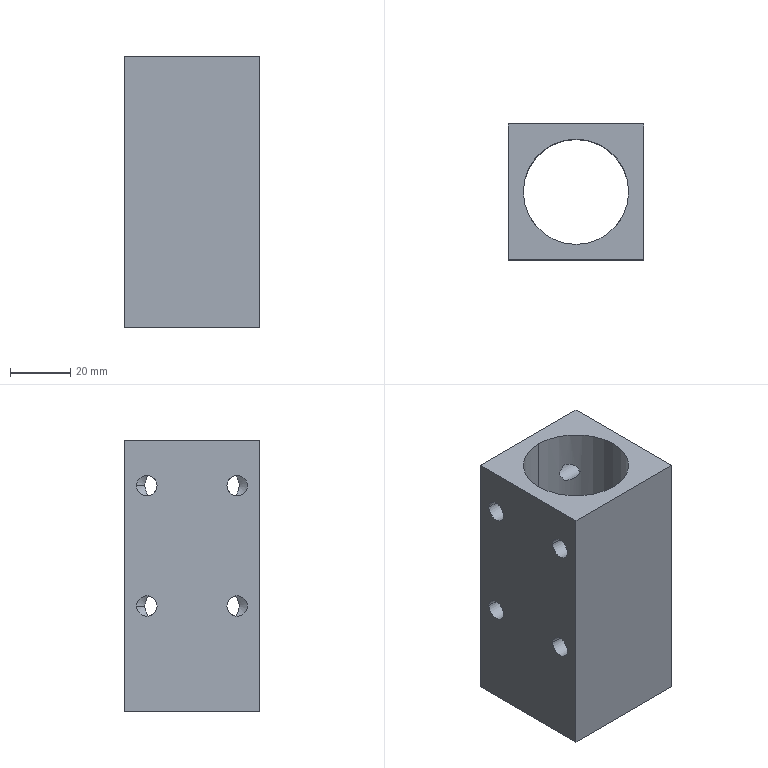Component | SolidWorks | UpperSideBeltXG-XG1-1_UpperSleeveXG-XG1-1 | 1 solid | 36 faces | box 45 x 45 x 90 mm | volume 92007 mm3 | cylinder 18 | cone 12 | plane 6 | commonest cylinder face diameters 6.8 x16 35 x2
build123d program:
from build123d import *

# Parameters (mm, degrees)
SKETCH1_W                  = 45
SKETCH1_H                  = 45
SKETCH1_R                  = 17.5
BOSS_EXTRUDE1_DEPTH        = 45
M8_TAPPED_HOLE1_AT_2_COUNT = 2
M8_TAPPED_HOLE1_AT_2_PITCH = 30
M8_TAPPED_HOLE1_AT_3_COUNT = 2
M8_TAPPED_HOLE1_AT_3_PITCH = 40
M8_TAPPED_HOLE1_AT_4_COUNT = 2
M8_TAPPED_HOLE1_AT_4_PITCH = 50


with BuildPart() as part:
    # Sketch1 → Boss-Extrude1 (new, symmetric)
    with BuildSketch(Plane(origin=(0, 0, 0), x_dir=(0, 0, -1), z_dir=(1, 0, 0))):
        Rectangle(SKETCH1_W, SKETCH1_H)
        with Locations(Location((0, 0, 0), (0, 0, 180))):
            Circle(SKETCH1_R, mode=Mode.SUBTRACT)
    extrude(amount=BOSS_EXTRUDE1_DEPTH, both=True)

    # Sketch2 → M8 Tapped Hole1 (revolve, cut)
    with BuildSketch(Plane(origin=(-30, -22.5, 15), x_dir=(0, 0, -1), z_dir=(1, 0, 0))):
        Polygon((0, 0), (0, 15.043), (3.4, 13), (3.4, 0), align=None)
    m8_tapped_hole1 = revolve(axis=Axis((-30, -28.85, 15), (0, 1, 0)), mode=Mode.SUBTRACT)

    # M8 Tapped Hole1 at 2: M8 Tapped Hole1 ×2
    with Locations(*[(0, 0, -i * M8_TAPPED_HOLE1_AT_2_PITCH) for i in range(1, M8_TAPPED_HOLE1_AT_2_COUNT)]):
        add(m8_tapped_hole1, mode=Mode.SUBTRACT)

    # M8 Tapped Hole1 at 3: M8 Tapped Hole1 ×2
    with Locations(*[(i * M8_TAPPED_HOLE1_AT_3_PITCH, 0, 0) for i in range(1, M8_TAPPED_HOLE1_AT_3_COUNT)]):
        add(m8_tapped_hole1, mode=Mode.SUBTRACT)

    # M8 Tapped Hole1 at 4: M8 Tapped Hole1 ×2
    with Locations(*[Vector(0.8, 0, -0.6) * (i * M8_TAPPED_HOLE1_AT_4_PITCH) for i in range(1, M8_TAPPED_HOLE1_AT_4_COUNT)]):
        add(m8_tapped_hole1, mode=Mode.SUBTRACT)

    # Mirror1: M8 Tapped Hole1 across plane
    add(m8_tapped_hole1.mirror(Plane.ZX), mode=Mode.SUBTRACT)

    # Mirror1 copy 1 sketch → Mirror1 copy 1 (revolve, cut)
    with BuildSketch(Plane(origin=(-30, 22.5, -15), x_dir=(0, 0, -1), z_dir=(1, 0, 0))):
        Polygon((0, 0), (0, -15.043), (3.4, -13), (3.4, 0), align=None)
    revolve(axis=Axis((-30, 28.85, -15), (0, 1, 0)), mode=Mode.SUBTRACT)

    # Mirror1 copy 2 sketch → Mirror1 copy 2 (revolve, cut)
    with BuildSketch(Plane(origin=(10, 22.5, 15), x_dir=(0, 0, -1), z_dir=(1, 0, 0))):
        Polygon((0, 0), (0, -15.043), (3.4, -13), (3.4, 0), align=None)
    revolve(axis=Axis((10, 28.85, 15), (0, 1, 0)), mode=Mode.SUBTRACT)

    # Mirror1 copy 3 sketch → Mirror1 copy 3 (revolve, cut)
    with BuildSketch(Plane(origin=(10, 22.5, -15), x_dir=(0, 0, -1), z_dir=(1, 0, 0))):
        Polygon((0, 0), (0, -15.043), (3.4, -13), (3.4, 0), align=None)
    revolve(axis=Axis((10, 28.85, -15), (0, 1, 0)), mode=Mode.SUBTRACT)


solid = part.part

# Placed as in the assembly
solid = solid.moved(Location((-348.72, 545, 263), (90, 0, -90)))